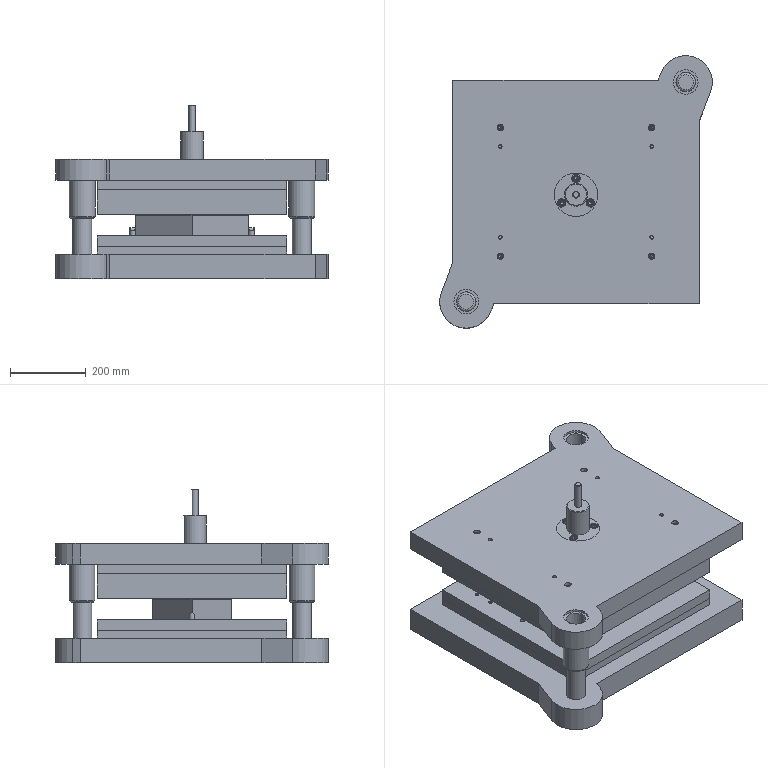Assembly | NX | mm | 47 component files | 47 solids | 787 faces | box 720 x 720 x 458 mm | volume 85015668 mm3 | plane 360 | cylinder 215 | cone 162 | torus 36 | spline 10 | other 4 | commonest cylinder face diameters 10 x44 12 x18 11 x16 9.732 x16 50 x12 8.06 x12 18 x9 16 x8
Bill of materials:
unnamed part 1 | 1 |  | Flanged cylindrical bushing: a thin round flange with a taller cylindrical boss on top and a central through bore.
GB-T70.1-2000,M10x70 | 4 |  | Hexagon Socket Head Cap Screw, GB-T 70.1-2000,M10x70
unnamed part 2 | 1 |  | Thin flat square plate with a pattern of small through holes and one larger central hole.
GB-T70.1-2000,M12x35 | 2 |  | Hexagon Socket Head Cap Screw, GB-T 70.1-2000,M12x35
GB-T70.1-2000,M20x140 | 1 |  | Hexagon Socket Head Cap Screw, GB-T 70.1-2000,M20x140
unnamed part 3 | 1 |  | Thin flat square plate with corner hole pairs and four pairs of holes placed in a cross pattern around the center.
unnamed part 4 | 1 |  | Thin flat circular disc with three large through holes evenly spaced around a small central hole.
GB-T70.1-2000,M10x100 | 4 |  | Hexagon Socket Head Cap Screw, GB-T 70.1-2000,M10x100
unnamed part 5 | 1 |  | Slender cylindrical pin with a short, smaller-diameter stepped end on one side.
unnamed part 6 | 1 |  | Thin flat square plate with corner hole pairs, a central hole, and four holes placed in a cross pattern around it.
unnamed part 7 | 4 |  | Stepped cylindrical pin with a thin head at one end, one or more larger-diameter sections, and a long smaller-diameter shank.
GB-T70.1-2000,M12x20 | 1 |  | Hexagon Socket Head Cap Screw, GB-T 70.1-2000,M12x20
unnamed part 8 | 1 |  | Thick square plate with a large pentagonal (arrow-shaped) through cutout and pairs of small holes near the corners.
unnamed part 9 | 2 |  | Hollow cylindrical sleeve with a stepped outer diameter: a smaller-diameter upper section and a larger-diameter lower section.
unnamed part 10 | 1 |  | Flat roughly square plate with two rounded lugs at opposite diagonal corners, each with a large hole, plus a central recess and a pattern of small holes.
unnamed part 11 | 4 |  | Slender plain cylindrical rod or pin with chamfered ends.
unnamed part 12 | 4 |  | Short solid cylindrical pin with chamfered ends.
unnamed part 13 | 1 |  | Thick plate shaped like a pentagon (house outline), with four small through holes near the vertices and a thin top layer that sticks out slightly past the body all the way around.
unnamed part 14 | 1 |  | Thin flat sheet with the same pentagonal outline and four small holes, with a raised flat-topped elliptical bulge in the middle that has rounded edges.
unnamed part 15 | 1 |  | Elliptical disc with a chamfered top edge and a small through hole in the center, a shorter cylindrical boss underneath, and a small hole drilled into the side.
unnamed part 16 | 1 |  | Square flat plate with two rounded tabs at opposite diagonal corners, each with a larger hole, and a regular pattern of smaller holes across the face.
unnamed part 17 | 1 |  | Thick pentagonal block with four small holes near the vertices and an elliptical shallow pocket in the middle, with a larger round through hole inside the pocket.
unnamed part 18 | 4 |  | Long, slender solid cylindrical rod with small chamfers on both ends.
unnamed part 19 | 2 |  | Solid cylindrical pin with rounded or chamfered edges at both ends; shorter and thicker than the slender rod.
unnamed part 20 | 2 |  | Stepped round pin: a larger cylindrical body ending in a two-faced wedge (chisel) tip, and a smaller-diameter shank on the other end with a narrow neck or groove next to the shoulder and a chamfered end.
Mates:
1. touch align | lower_die_base 1 datumplane | assembly datumplane
2. touch align | lower_die_base 1 datumplane | assembly datumplane
3. touch align | lower_die_base 1 face | assembly datumplane
4. center | spacer_plate 1 face | spacer_plate 1 face | lower_die_base 1 face | lower_die_base 1 face
5. center | spacer_plate 1 face | spacer_plate 1 face | lower_die_base 1 face | lower_die_base 1 face
6. touch align | spacer_plate 1 face | lower_die_base 1 face
7. center | die_fix_plate 1 face | die_fix_plate 1 face | spacer_plate 1 face | spacer_plate 1 face
8. center | die_fix_plate 1 face | die_fix_plate 1 face | spacer_plate 1 face | spacer_plate 1 face
9. touch align | die_fix_plate 1 face | spacer_plate 1 face
10. center | trim_punch_die 1 face | trim_punch_die 1 face | die_fix_plate 1 face | die_fix_plate 1 face
11. touch align | trim_punch_die 1 face | die_fix_plate 1 face
12. align lock | trim_punch_die 1 face | spacer_plate 1 face
13. touch align | locating_block 1 face | trim_punch_die 1 face
14. align lock | locating_block 1 face | trim_punch_die 1 face
15. touch align | drawn_part 1 face | locating_block 1 face
16. touch align | drawn_part 1 | locating_block 1
17. touch align | ejector_block 1 | locating_block 1
18. touch align | ejector_block 1 | locating_block 1
19. touch align | ejector_block 1 face | drawn_part 1 face
20. touch align | die 1 datumplane | ejector_block 1
21. touch align | die 1 datumplane | ejector_block 1
22. touch align | die 1 face | ejector_block 1 face
23. center | punch_fix_plate 1 face | punch_fix_plate 1 face | die 1 face | die 1 face
24. center | punch_fix_plate 1 face | punch_fix_plate 1 face | die 1 face | die 1 face
25. center | upper_die_base 1 face | upper_die_base 1 face | lower_die_base 1 face | lower_die_base 1 face
26. center | upper_die_base 1 face | upper_die_base 1 face | lower_die_base 1 face | lower_die_base 1 face
27. touch align | punch_fix_plate 1 face | die 1 face
28. concentric | die_shank 1 edge | upper_die_base 1 edge
29. concentric | die_shank 1 edge | upper_die_base 1 edge
30. touch align | upper_die_base 1 face | punch_fix_plate 1 face
31. concentric | outer_guide_bush 1 edge | upper_die_base 1 edge
32. concentric | outer_guide_bush 2 edge | upper_die_base 1 edge
33. align lock | outer_guide_post 1 face | outer_guide_bush 2 face
34. align lock | outer_guide_post 2 face | outer_guide_bush 1 face
35. distance | outer_guide_post 2 face | lower_die_base 1 face
36. distance | outer_guide_post 1 face | lower_die_base 1 face
37. align lock | dowel_pin_100 4 face | lower_die_base 1 face
38. align lock | dowel_pin_100 2 face | lower_die_base 1 face
39. align lock | dowel_pin_100 3 face | lower_die_base 1 face
40. align lock | dowel_pin_100 1 face | lower_die_base 1 face
41. distance | dowel_pin_100 4 face | lower_die_base 1 face
42. distance | dowel_pin_100 2 face | lower_die_base 1 face
43. distance | dowel_pin_100 3 face | lower_die_base 1 face
44. distance | dowel_pin_100 1 face | lower_die_base 1 face
45. align lock | dowel_pin_130 1 face | upper_die_base 1 face
46. align lock | dowel_pin_130 2 face | upper_die_base 1 face
47. align lock | dowel_pin_130 3 face | upper_die_base 1 face
48. align lock | dowel_pin_130 4 face | upper_die_base 1 face
49. distance | dowel_pin_130 3 face | upper_die_base 1 face
50. distance | dowel_pin_130 4 face | upper_die_base 1 face
51. distance | dowel_pin_130 2 face | upper_die_base 1 face
52. distance | dowel_pin_130 1 face | upper_die_base 1 face